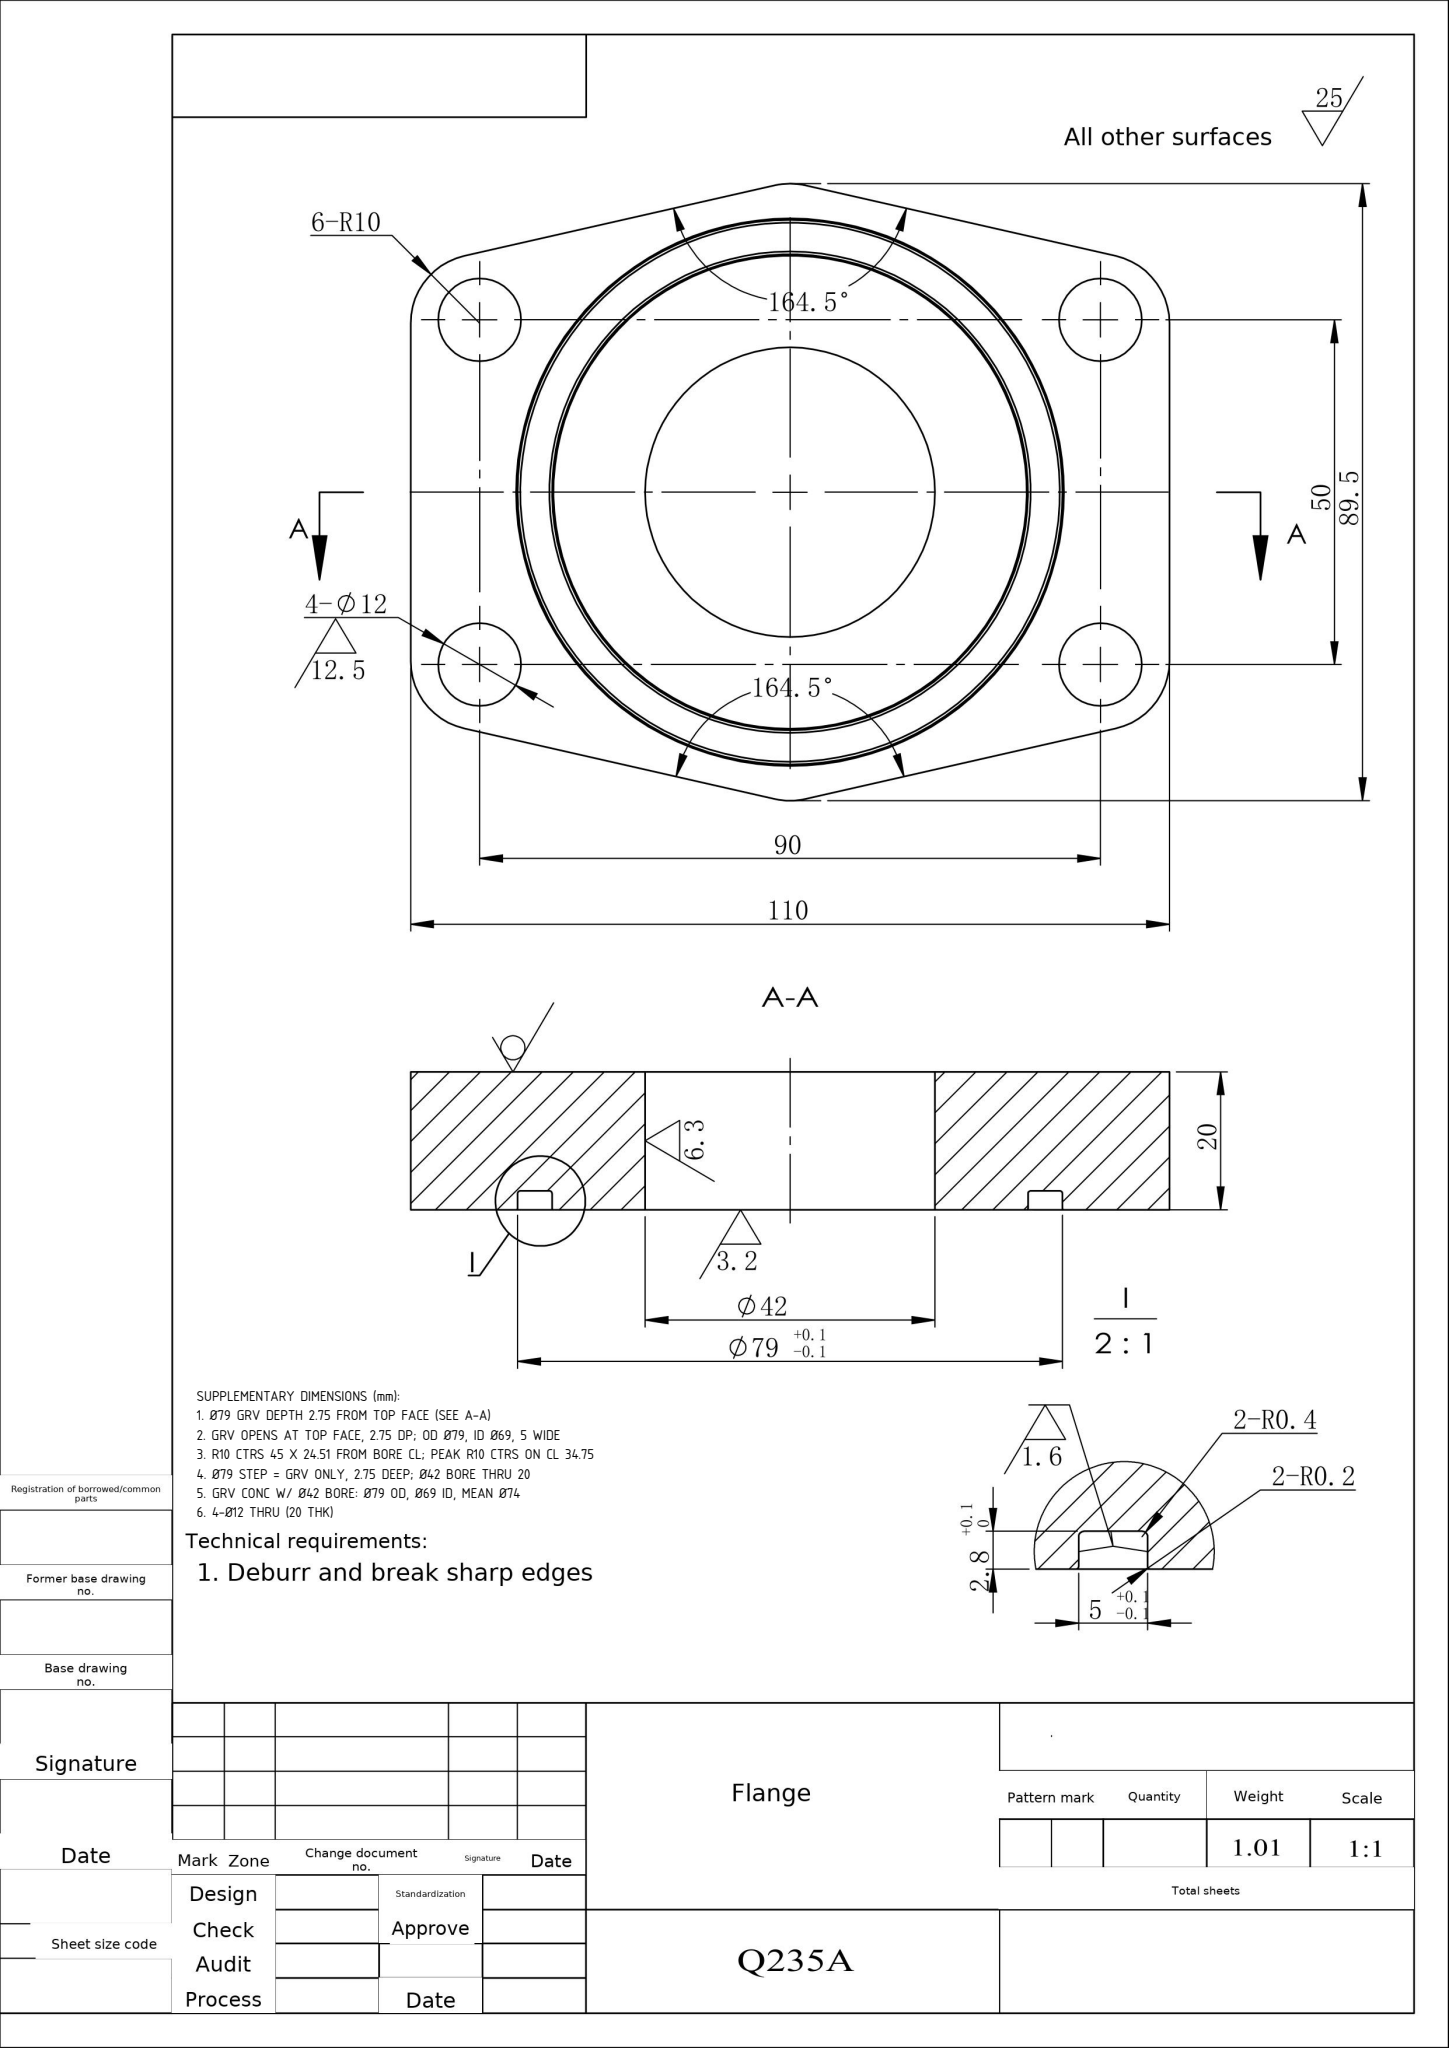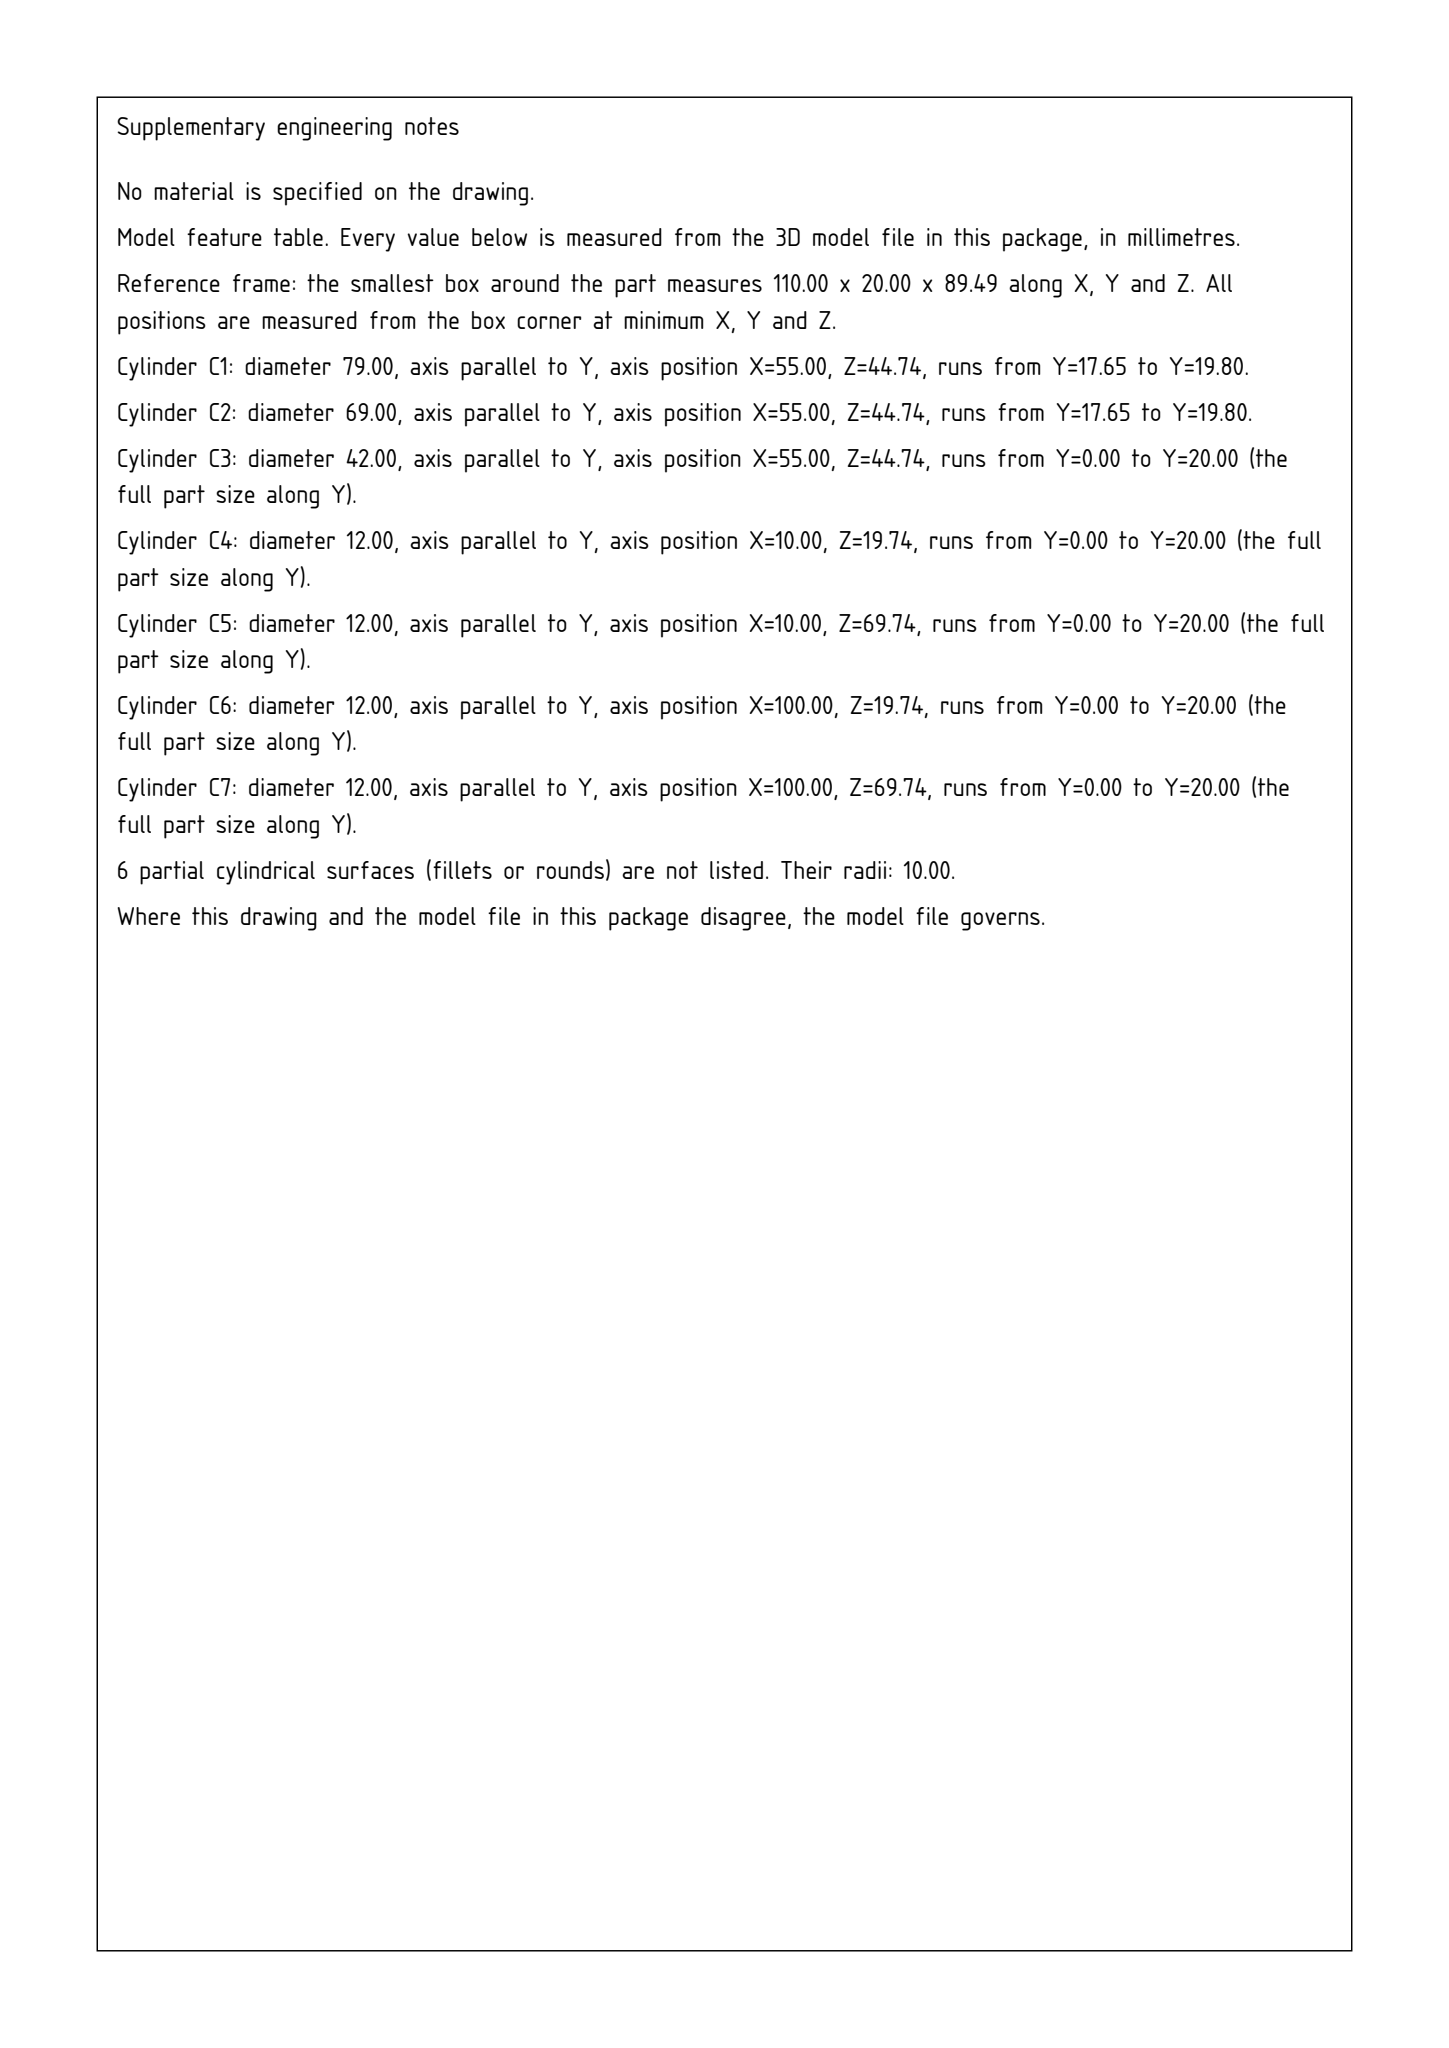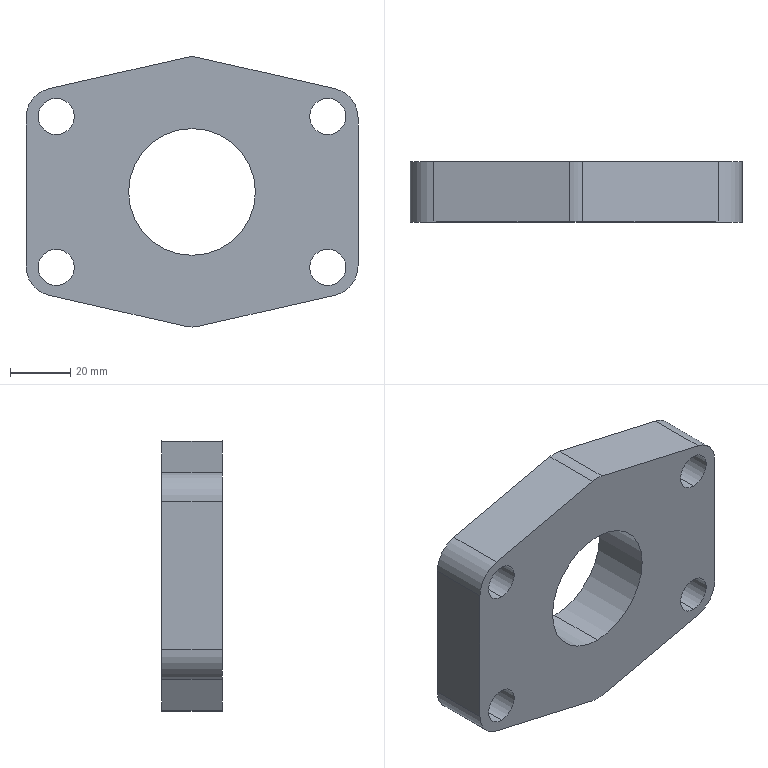Part | SolidWorks | mm | 1 solid | 39 faces | box 110 x 20 x 89.49 mm | volume 129547 mm3 | cylinder 21 | plane 10 | torus 8 | commonest cylinder face diameters 12 x8 20 x7 69 x2 79 x2 42 x2
build123d program:
from build123d import *

# Parameters (mm, degrees)
SKETCH1_R           = 6
SKETCH1_R_2         = 21
BOSS_EXTRUDE1_DEPTH = 20
FILLET1_R           = 10
SKETCH3_R           = 39.5
SKETCH3_R_2         = 34.5
CUT_EXTRUDE2_DEPTH  = 2.75
FILLET8_R           = 0.4
FILLET9_R           = 0.2


with BuildPart() as part:
    # Sketch1 → Boss-Extrude1 (new body)
    with BuildSketch(Plane(origin=(0, 0, 0), x_dir=(1, 0, 0), z_dir=(0, 1, 0))):
        Polygon((0, 45), (-55, 32.5), (-55, -32.5), (0, -45), (55, -32.5), (55, 32.5), align=None)
        with Locations(Location((45, 25, 0), (0, 0, 270))):
            Circle(SKETCH1_R, mode=Mode.SUBTRACT)
        with Locations(Location((45, -25, 0), (0, 0, 270))):
            Circle(SKETCH1_R, mode=Mode.SUBTRACT)
        with Locations(Location((-45, 25, 0), (0, 0, 270))):
            Circle(SKETCH1_R, mode=Mode.SUBTRACT)
        with Locations(Location((-45, -25, 0), (0, 0, 270))):
            Circle(SKETCH1_R, mode=Mode.SUBTRACT)
        with Locations(Location((0, 0, 0), (0, 0, 270))):
            Circle(SKETCH1_R_2, mode=Mode.SUBTRACT)
    extrude(amount=BOSS_EXTRUDE1_DEPTH)

    # Fillet1
    fillet1_edges = [part.edges().sort_by_distance(p)[0] for p in [
        (55, 10, -32.5),
        (55, 10, 32.5),
        (0, 10, 45),
        (-55, 10, 32.5),
        (-55, 10, -32.5),
        (0, 10, -45),
    ]]
    fillet(fillet1_edges, radius=FILLET1_R)

    # Sketch3 → Cut-Extrude2 (cut)
    with BuildSketch(Plane(origin=(0, 20, 0), x_dir=(1, 0, 0), z_dir=(0, 1, 0))):
        with Locations(Location((0, 0, 0), (0, 0, 270))):
            Circle(SKETCH3_R)
        with Locations(Location((0, 0, 0), (0, 0, 270))):
            Circle(SKETCH3_R_2, mode=Mode.SUBTRACT)
    extrude(amount=-CUT_EXTRUDE2_DEPTH, mode=Mode.SUBTRACT)

    # Fillet8
    fillet8_edges = [part.edges().sort_by_distance(p)[0] for p in [
        (0, 17.25, -39.5),
        (0, 17.25, -34.5),
    ]]
    fillet(fillet8_edges, radius=FILLET8_R)

    # Fillet9
    fillet9_edges = [part.edges().sort_by_distance(p)[0] for p in [
        (0, 20, -39.5),
        (0, 20, -34.5),
    ]]
    fillet(fillet9_edges, radius=FILLET9_R)


solid = part.part